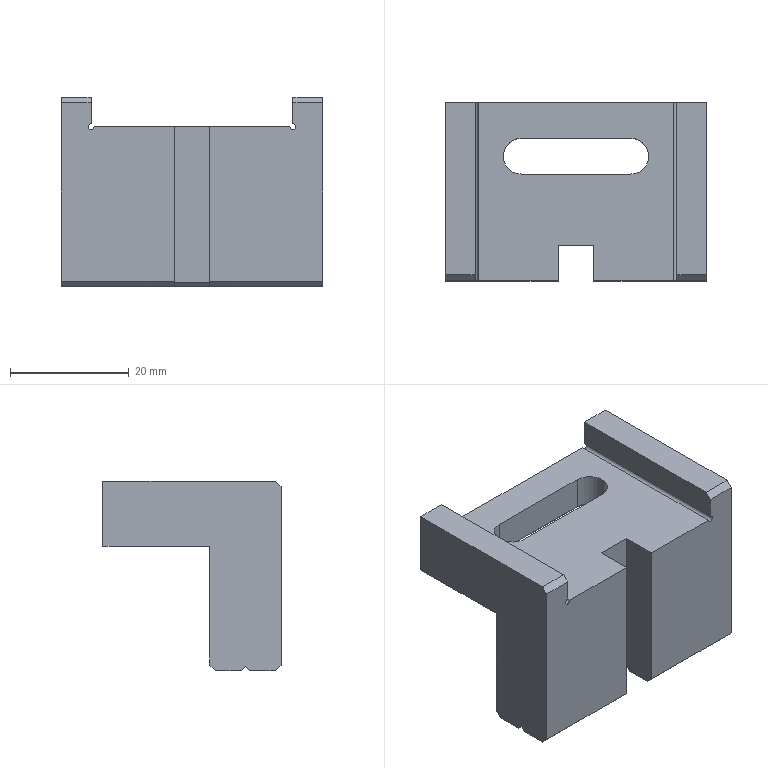Component | NX | GUIDE_BLOCK | 1 solid | 36 faces | volume 18594 mm3 | plane 30 | cylinder 4 | cone 2 | commonest cylinder face diameters 1 x2 6 x2